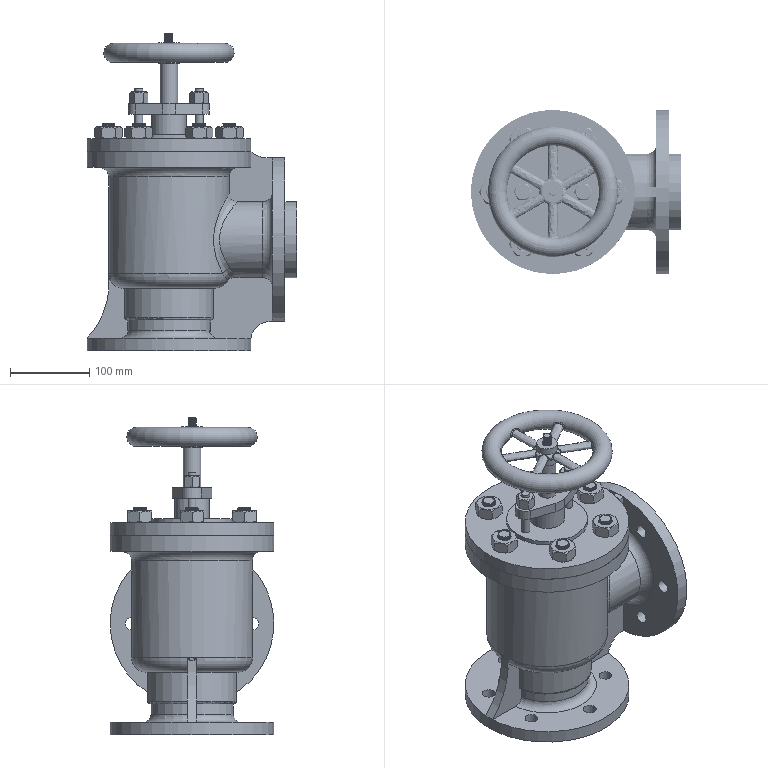Assembly | NX | mm | 23 component files | 26 solids | 561 faces | box 264 x 206 x 400 mm | volume 4348735 mm3 | cylinder 255 | plane 176 | spline 69 | cone 31 | torus 24 | other 6 | commonest cylinder face diameters 16 x174 14 x12 10 x9 17 x6 206 x5 22 x4 96 x4 26 x4
Bill of materials:
unnamed part 1 | 1 |  | Circular flange plate with a central hub and a downward-tapering conical stem; the plate has a ring of six through holes, a central bore and two small holes near the center.
unnamed part 2 | 1 |  | Diamond/oval two-hole flange with a cylindrical spigot body and a central through bore.
unnamed part 3 | 1 |  | Circular cap/disc head with a small raised center boss on top and a body of intersecting flat plates (cross-shaped legs) below.
unnamed part 4 | 6 |  | Cylindrical stud with modeled external threads on both ends and a plain unthreaded middle section.
unnamed part 5 | 6 |  | Hexagonal nut with a modeled internal thread and chamfered corners on both faces.
unnamed part 6 | 1 |  | Spoked handwheel: toroidal rim joined by six radial spokes to a central cylindrical hub with a bore.
unnamed part 7 | 1 |  | Flanged tee-type body: a main cylindrical body with circular bolted flanges at both ends and a side branch ending in its own bolted flange.
unnamed part 8 | 2 |  | Plain solid cylindrical rod or pin with flat ends.
unnamed part 9 | 1 |  | Thin-walled flanged cylindrical sleeve/bushing with a through bore.
unnamed part 10 | 1 |  | Long stepped shaft with a short collar/head at one end, a threaded section next to the collar, a long plain shank, and a reduced-diameter neck ending in a small threaded tip.
unnamed part 11 | 2 |  | Hexagonal nut, taller relative to its width, with a modeled internal thread and chamfered corners on both faces.
Mates:
1. touch align | 03__Hand_Wheel__2 1 face | 07__Spindle__2 1 face
2. concentric | 03__Hand_Wheel__2 1 edge | 07__Spindle__2 1 edge
3. touch align | 06__Gland__2 1 face | 07__Spindle__2 1 face
4. touch align | 07__Spindle__2 1 face | 01__Body__2 1 face
5. concentric | 05__Valve__2 1 edge | 07__Spindle__2 1 edge
6. touch align | 04__Valve_Seat__2 1 face | 07__Spindle__2 1 face
7. concentric | 04__Valve_Seat__2 1 edge | 01__Body__2 1 edge
8. touch align | 08__Stud_M10x1__2 2 face | 06__Gland__2 1 face
9. fix | assembly component
10. bond | 09__Stud_M16x1_5__2 6 component | assembly component
11. bond | 09__Stud_M16x1_5__2 5 component | assembly component
12. bond | 09__Stud_M16x1_5__2 4 component | assembly component
13. bond | 09__Stud_M16x1_5__2 3 component | assembly component
14. bond | 09__Stud_M16x1_5__2 2 component | assembly component
15. bond | 09__Stud_M16x1_5__2 1 component | assembly component
16. circular | assembly datumaxis | assembly cartesiancoordinatesystem | assembly cartesiancoordinatesystem | assembly cartesiancoordinatesystem | assembly cartesiancoordinatesystem | assembly cartesiancoordinatesystem | assembly cartesiancoordinatesystem
17. fix | assembly component
18. bond | 08__Stud_M10x1__2 2 component | assembly component
19. bond | 08__Stud_M10x1__2 1 component | assembly component
20. circular | assembly datumaxis | assembly cartesiancoordinatesystem | assembly cartesiancoordinatesystem
21. touch align | 10__Nut_M16x1_5__2 6 face | 09__Stud_M16x1_5__2 6 face
22. touch align | 11__Nut_M10x1__2 2 face | 08__Stud_M10x1__2 2 face
23. touch align | 11__Nut_M10x1__2 2 face | 06__Gland__2 1 face
24. bond | 06__Gland__2 1 component | assembly component
25. bond | 11__Nut_M10x1__2 2 component | assembly component
26. bond | 11__Nut_M10x1__2 1 component | assembly component
27. circular | assembly datumaxis | assembly cartesiancoordinatesystem | assembly cartesiancoordinatesystem
28. bond | 06__Gland__2 1 component | assembly component
29. bond | 10__Nut_M16x1_5__2 6 component | assembly component
30. bond | 10__Nut_M16x1_5__2 5 component | assembly component
31. bond | 10__Nut_M16x1_5__2 4 component | assembly component
32. bond | 10__Nut_M16x1_5__2 3 component | assembly component
33. bond | 10__Nut_M16x1_5__2 2 component | assembly component
34. bond | 10__Nut_M16x1_5__2 1 component | assembly component
35. circular | assembly datumaxis | assembly cartesiancoordinatesystem | assembly cartesiancoordinatesystem | assembly cartesiancoordinatesystem | assembly cartesiancoordinatesystem | assembly cartesiancoordinatesystem | assembly cartesiancoordinatesystem
36. touch align | 02__Cover__2 1 face | 06__Gland__2 1 face
37. touch align | 02__Cover__2 1 face | 09__Stud_M16x1_5__2 6 face
38. touch align | 09__Stud_M16x1_5__2 1 face | 02__Cover__2 1 face
39. touch align | 09__Stud_M16x1_5__2 2 face | 02__Cover__2 1 face
40. touch align | 02__Cover__2 1 face | 01__Body__2 1 face
41. concentric | 01__Body__2 1 edge | 09__Stud_M16x1_5__2 6 edge